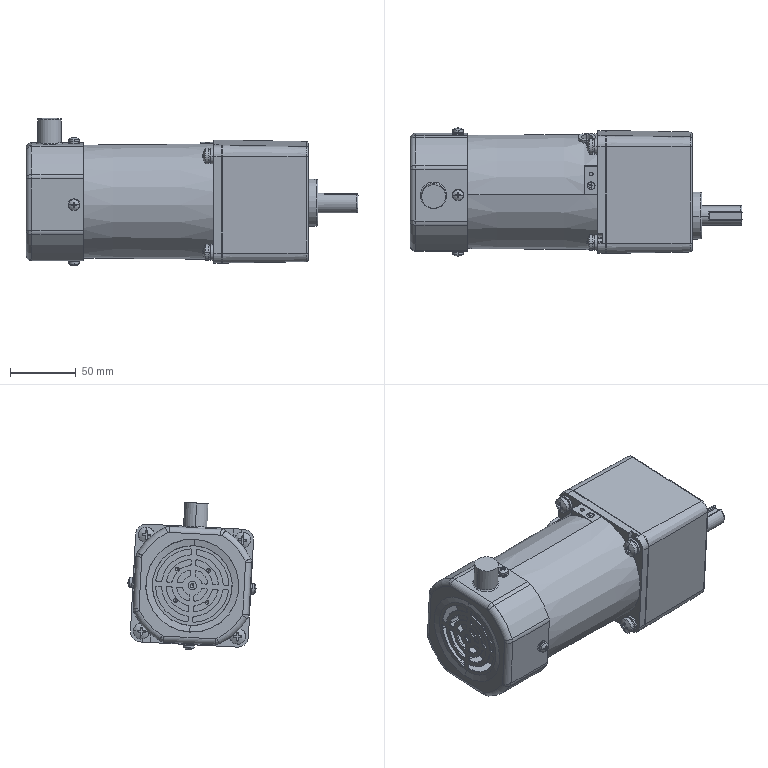Component | SolidWorks | StepperMotor-2 | 23 solids | 830 faces | volume 1251545 mm3 | cylinder 382 | plane 307 | cone 53 | torus 48 | sphere 22 | spline 18 | commonest cylinder face diameters 2 x53 0.6 x32 12 x22 9 x16 4 x16 4.4 x16 6.6 x16 6.68 x13